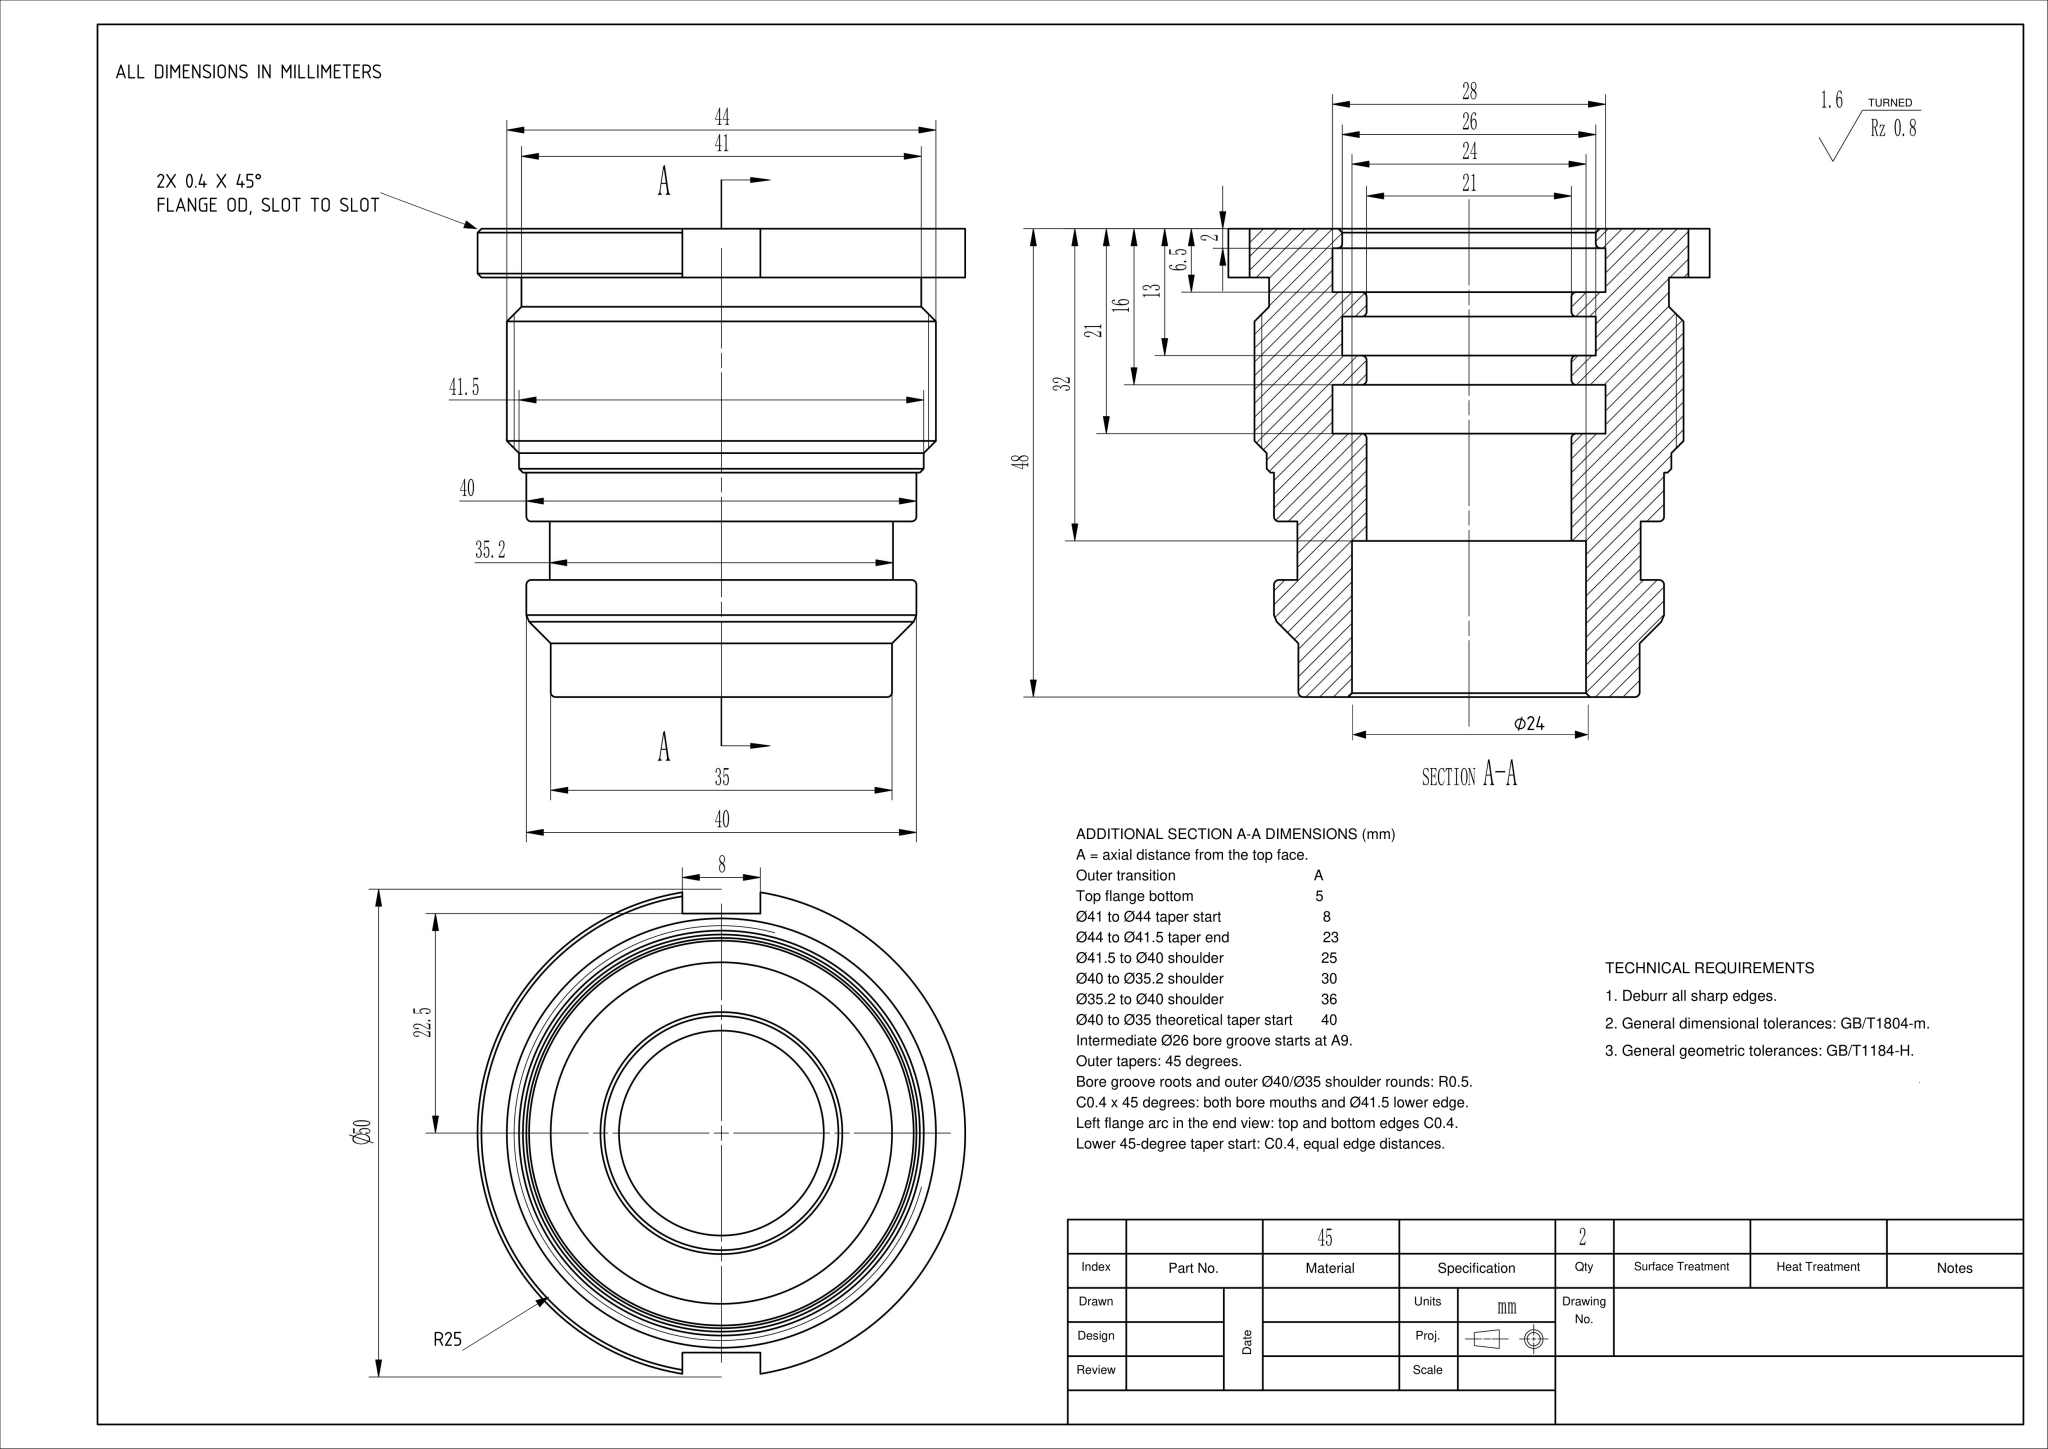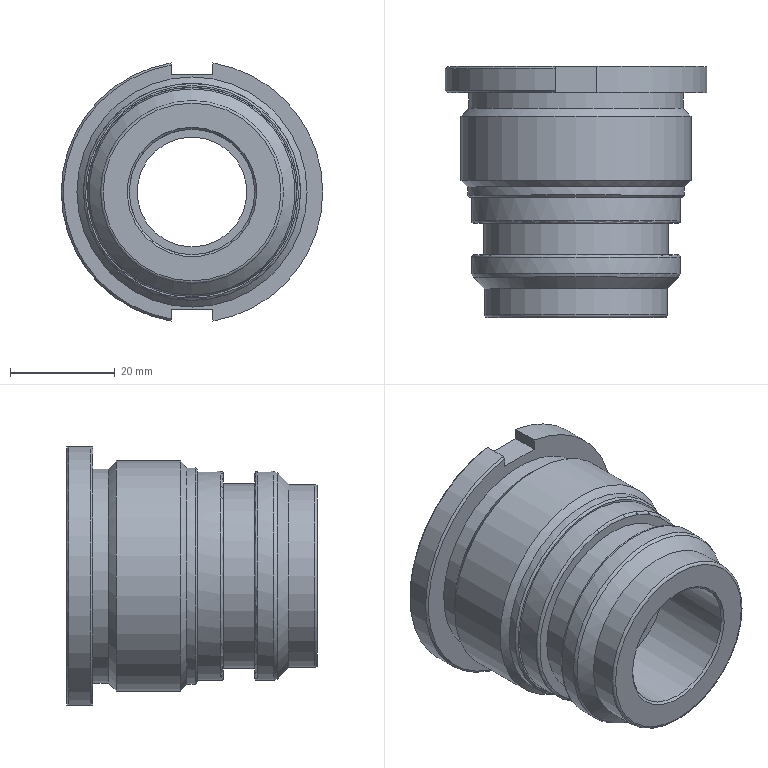Part | NX | mm | 1 solid | 54 faces | box 50 x 48 x 49.36 mm | volume 41976 mm3 | plane 19 | cylinder 17 | cone 9 | torus 9 | commonest cylinder face diameters 21 x3 50 x2 26 x2 28 x2 40 x2 41 x1 44 x1 41.5 x1